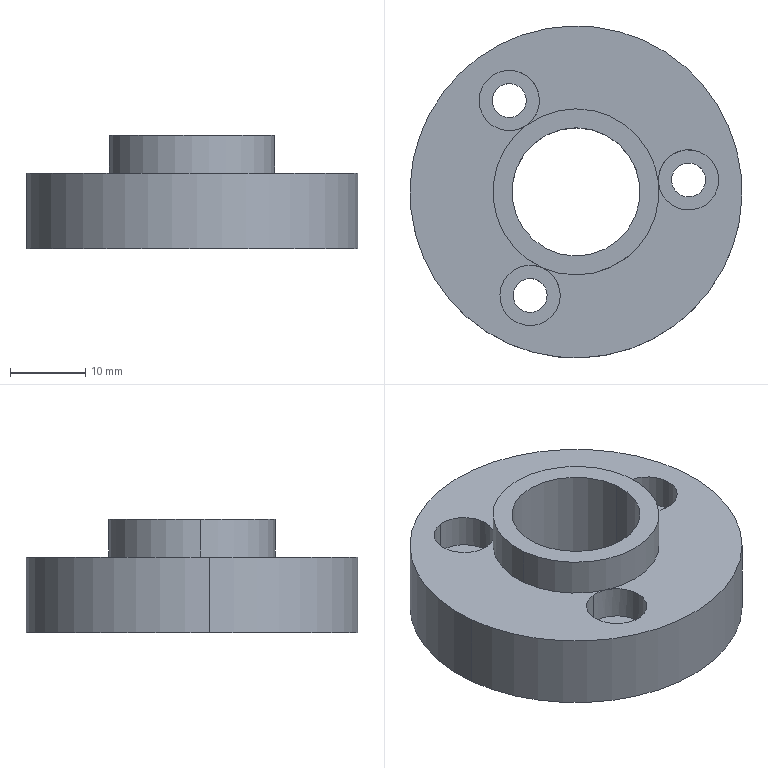Component | SolidWorks | XT-1-15-2-2 | 1 solid | 24 faces | box 44 x 44 x 15 mm | volume 12771 mm3 | cylinder 18 | plane 6 | commonest cylinder face diameters 8 x6 4.5 x6 17 x2 22 x2 44 x2
STEP:
#1=COLOUR_RGB('',0.7922,0.8196,0.9333);
#2=FILL_AREA_STYLE_COLOUR('',#1);
#3=FILL_AREA_STYLE('',(#2));
#4=SURFACE_STYLE_FILL_AREA(#3);
#5=SURFACE_SIDE_STYLE('',(#4));
#6=SURFACE_STYLE_USAGE(.BOTH.,#5);
#7=PRESENTATION_STYLE_ASSIGNMENT((#6));
#8=CARTESIAN_POINT('',(19.42,-9.62,-0.05512));
#9=VERTEX_POINT('',#8);
#10=CARTESIAN_POINT('',(19.454,-9.933,-0.05512));
#11=VERTEX_POINT('',#10);
#12=CARTESIAN_POINT('',(19.437,-9.777,-0.05512));
#13=DIRECTION('',(-0.,-0.,1.));
#14=DIRECTION('',(0.1062,-0.9943,-0.));
#15=AXIS2_PLACEMENT_3D('',#12,#13,#14);
#16=CIRCLE('',#15,0.1575);
#17=EDGE_CURVE('',#9,#11,#16,.T.);
#18=ORIENTED_EDGE('',*,*,#17,.F.);
#19=CARTESIAN_POINT('',(19.42,-9.62,0.1181));
#20=VERTEX_POINT('',#19);
#21=CARTESIAN_POINT('',(19.42,-9.62,0.1181));
#22=DIRECTION('',(-0.,-0.,1.));
#23=VECTOR('',#22,39.37);
#24=LINE('',#21,#23);
#25=EDGE_CURVE('',#9,#20,#24,.T.);
#26=ORIENTED_EDGE('',*,*,#25,.T.);
#27=CARTESIAN_POINT('',(19.454,-9.933,0.1181));
#28=VERTEX_POINT('',#27);
#29=CARTESIAN_POINT('',(19.437,-9.777,0.1181));
#30=DIRECTION('',(-0.,-0.,1.));
#31=DIRECTION('',(0.1062,-0.9943,-0.));
#32=AXIS2_PLACEMENT_3D('',#29,#30,#31);
#33=CIRCLE('',#32,0.1575);
#34=EDGE_CURVE('',#20,#28,#33,.T.);
#35=ORIENTED_EDGE('',*,*,#34,.T.);
#36=CARTESIAN_POINT('',(19.454,-9.933,0.1181));
#37=DIRECTION('',(-0.,-0.,1.));
#38=VECTOR('',#37,39.37);
#39=LINE('',#36,#38);
#40=EDGE_CURVE('',#11,#28,#39,.T.);
#41=ORIENTED_EDGE('',*,*,#40,.F.);
#42=EDGE_LOOP('',(#18,#26,#35,#41));
#43=FACE_OUTER_BOUND('',#42,.T.);
#44=CARTESIAN_POINT('',(19.437,-9.777,0.1181));
#45=DIRECTION('',(-0.,-0.,1.));
#46=DIRECTION('',(0.1062,-0.9943,-0.));
#47=AXIS2_PLACEMENT_3D('',#44,#45,#46);
#48=CYLINDRICAL_SURFACE('',#47,0.1575);
#49=ADVANCED_FACE('',(#43),#48,.F.);
#50=CARTESIAN_POINT('',(19.428,-9.689,-0.2756));
#51=VERTEX_POINT('',#50);
#52=CARTESIAN_POINT('',(19.447,-9.865,-0.2756));
#53=VERTEX_POINT('',#52);
#54=CARTESIAN_POINT('',(19.437,-9.777,-0.2756));
#55=DIRECTION('',(-0.,-0.,1.));
#56=DIRECTION('',(0.1062,-0.9943,0.));
#57=AXIS2_PLACEMENT_3D('',#54,#55,#56);
#58=CIRCLE('',#57,0.08858);
#59=EDGE_CURVE('',#51,#53,#58,.T.);
#60=ORIENTED_EDGE('',*,*,#59,.F.);
#61=CARTESIAN_POINT('',(19.428,-9.689,-0.05512));
#62=VERTEX_POINT('',#61);
#63=CARTESIAN_POINT('',(19.428,-9.689,0.1181));
#64=DIRECTION('',(-0.,-0.,1.));
#65=VECTOR('',#64,39.37);
#66=LINE('',#63,#65);
#67=EDGE_CURVE('',#51,#62,#66,.T.);
#68=ORIENTED_EDGE('',*,*,#67,.T.);
#69=CARTESIAN_POINT('',(19.447,-9.865,-0.05512));
#70=VERTEX_POINT('',#69);
#71=CARTESIAN_POINT('',(19.437,-9.777,-0.05512));
#72=DIRECTION('',(-0.,-0.,1.));
#73=DIRECTION('',(0.1062,-0.9943,-0.));
#74=AXIS2_PLACEMENT_3D('',#71,#72,#73);
#75=CIRCLE('',#74,0.08858);
#76=EDGE_CURVE('',#62,#70,#75,.T.);
#77=ORIENTED_EDGE('',*,*,#76,.T.);
#78=CARTESIAN_POINT('',(19.447,-9.865,0.1181));
#79=DIRECTION('',(-0.,-0.,1.));
#80=VECTOR('',#79,39.37);
#81=LINE('',#78,#80);
#82=EDGE_CURVE('',#53,#70,#81,.T.);
#83=ORIENTED_EDGE('',*,*,#82,.F.);
#84=EDGE_LOOP('',(#60,#68,#77,#83));
#85=FACE_OUTER_BOUND('',#84,.T.);
#86=CARTESIAN_POINT('',(19.437,-9.777,0.1181));
#87=DIRECTION('',(-0.,-0.,1.));
#88=DIRECTION('',(0.1062,-0.9943,0.));
#89=AXIS2_PLACEMENT_3D('',#86,#87,#88);
#90=CYLINDRICAL_SURFACE('',#89,0.08858);
#91=ADVANCED_FACE('',(#85),#90,.F.);
#92=CARTESIAN_POINT('',(19.312,-8.603,-0.05512));
#93=VERTEX_POINT('',#92);
#94=CARTESIAN_POINT('',(19.345,-8.916,-0.05512));
#95=VERTEX_POINT('',#94);
#96=CARTESIAN_POINT('',(19.329,-8.76,-0.05512));
#97=DIRECTION('',(-0.,-0.,1.));
#98=DIRECTION('',(0.1062,-0.9943,-0.));
#99=AXIS2_PLACEMENT_3D('',#96,#97,#98);
#100=CIRCLE('',#99,0.1575);
#101=EDGE_CURVE('',#93,#95,#100,.T.);
#102=ORIENTED_EDGE('',*,*,#101,.F.);
#103=CARTESIAN_POINT('',(19.312,-8.603,0.1181));
#104=VERTEX_POINT('',#103);
#105=CARTESIAN_POINT('',(19.312,-8.603,0.1181));
#106=DIRECTION('',(-0.,-0.,1.));
#107=VECTOR('',#106,39.37);
#108=LINE('',#105,#107);
#109=EDGE_CURVE('',#93,#104,#108,.T.);
#110=ORIENTED_EDGE('',*,*,#109,.T.);
#111=CARTESIAN_POINT('',(19.345,-8.916,0.1181));
#112=VERTEX_POINT('',#111);
#113=CARTESIAN_POINT('',(19.329,-8.76,0.1181));
#114=DIRECTION('',(-0.,-0.,1.));
#115=DIRECTION('',(0.1062,-0.9943,-0.));
#116=AXIS2_PLACEMENT_3D('',#113,#114,#115);
#117=CIRCLE('',#116,0.1575);
#118=EDGE_CURVE('',#104,#112,#117,.T.);
#119=ORIENTED_EDGE('',*,*,#118,.T.);
#120=CARTESIAN_POINT('',(19.345,-8.916,0.1181));
#121=DIRECTION('',(-0.,-0.,1.));
#122=VECTOR('',#121,39.37);
#123=LINE('',#120,#122);
#124=EDGE_CURVE('',#95,#112,#123,.T.);
#125=ORIENTED_EDGE('',*,*,#124,.F.);
#126=EDGE_LOOP('',(#102,#110,#119,#125));
#127=FACE_OUTER_BOUND('',#126,.T.);
#128=CARTESIAN_POINT('',(19.329,-8.76,0.1181));
#129=DIRECTION('',(-0.,-0.,1.));
#130=DIRECTION('',(0.1062,-0.9943,-0.));
#131=AXIS2_PLACEMENT_3D('',#128,#129,#130);
#132=CYLINDRICAL_SURFACE('',#131,0.1575);
#133=ADVANCED_FACE('',(#127),#132,.F.);
#134=CARTESIAN_POINT('',(19.319,-8.672,-0.2756));
#135=VERTEX_POINT('',#134);
#136=CARTESIAN_POINT('',(19.338,-8.848,-0.2756));
#137=VERTEX_POINT('',#136);
#138=CARTESIAN_POINT('',(19.329,-8.76,-0.2756));
#139=DIRECTION('',(-0.,-0.,1.));
#140=DIRECTION('',(0.1062,-0.9943,0.));
#141=AXIS2_PLACEMENT_3D('',#138,#139,#140);
#142=CIRCLE('',#141,0.08858);
#143=EDGE_CURVE('',#135,#137,#142,.T.);
#144=ORIENTED_EDGE('',*,*,#143,.F.);
#145=CARTESIAN_POINT('',(19.319,-8.672,-0.05512));
#146=VERTEX_POINT('',#145);
#147=CARTESIAN_POINT('',(19.319,-8.672,0.1181));
#148=DIRECTION('',(-0.,-0.,1.));
#149=VECTOR('',#148,39.37);
#150=LINE('',#147,#149);
#151=EDGE_CURVE('',#135,#146,#150,.T.);
#152=ORIENTED_EDGE('',*,*,#151,.T.);
#153=CARTESIAN_POINT('',(19.338,-8.848,-0.05512));
#154=VERTEX_POINT('',#153);
#155=CARTESIAN_POINT('',(19.329,-8.76,-0.05512));
#156=DIRECTION('',(-0.,-0.,1.));
#157=DIRECTION('',(0.1062,-0.9943,-0.));
#158=AXIS2_PLACEMENT_3D('',#155,#156,#157);
#159=CIRCLE('',#158,0.08858);
#160=EDGE_CURVE('',#146,#154,#159,.T.);
#161=ORIENTED_EDGE('',*,*,#160,.T.);
#162=CARTESIAN_POINT('',(19.338,-8.848,0.1181));
#163=DIRECTION('',(-0.,-0.,1.));
#164=VECTOR('',#163,39.37);
#165=LINE('',#162,#164);
#166=EDGE_CURVE('',#137,#154,#165,.T.);
#167=ORIENTED_EDGE('',*,*,#166,.F.);
#168=EDGE_LOOP('',(#144,#152,#161,#167));
#169=FACE_OUTER_BOUND('',#168,.T.);
#170=CARTESIAN_POINT('',(19.329,-8.76,0.1181));
#171=DIRECTION('',(-0.,-0.,1.));
#172=DIRECTION('',(0.1062,-0.9943,-0.));
#173=AXIS2_PLACEMENT_3D('',#170,#171,#172);
#174=CYLINDRICAL_SURFACE('',#173,0.08858);
#175=ADVANCED_FACE('',(#169),#174,.F.);
#176=CARTESIAN_POINT('',(20.247,-9.018,-0.05512));
#177=VERTEX_POINT('',#176);
#178=CARTESIAN_POINT('',(20.28,-9.331,-0.05512));
#179=VERTEX_POINT('',#178);
#180=CARTESIAN_POINT('',(20.264,-9.174,-0.05512));
#181=DIRECTION('',(-0.,-0.,1.));
#182=DIRECTION('',(0.1062,-0.9943,-0.));
#183=AXIS2_PLACEMENT_3D('',#180,#181,#182);
#184=CIRCLE('',#183,0.1575);
#185=EDGE_CURVE('',#177,#179,#184,.T.);
#186=ORIENTED_EDGE('',*,*,#185,.F.);
#187=CARTESIAN_POINT('',(20.247,-9.018,0.1181));
#188=VERTEX_POINT('',#187);
#189=CARTESIAN_POINT('',(20.247,-9.018,0.1181));
#190=DIRECTION('',(-0.,-0.,1.));
#191=VECTOR('',#190,39.37);
#192=LINE('',#189,#191);
#193=EDGE_CURVE('',#177,#188,#192,.T.);
#194=ORIENTED_EDGE('',*,*,#193,.T.);
#195=CARTESIAN_POINT('',(20.107,-9.191,0.1181));
#196=VERTEX_POINT('',#195);
#197=CARTESIAN_POINT('',(20.264,-9.174,0.1181));
#198=DIRECTION('',(-0.,-0.,1.));
#199=DIRECTION('',(0.1062,-0.9943,-0.));
#200=AXIS2_PLACEMENT_3D('',#197,#198,#199);
#201=CIRCLE('',#200,0.1575);
#202=EDGE_CURVE('',#188,#196,#201,.T.);
#203=ORIENTED_EDGE('',*,*,#202,.T.);
#204=CARTESIAN_POINT('',(20.28,-9.331,0.1181));
#205=VERTEX_POINT('',#204);
#206=CARTESIAN_POINT('',(20.264,-9.174,0.1181));
#207=DIRECTION('',(-0.,-0.,1.));
#208=DIRECTION('',(0.1062,-0.9943,-0.));
#209=AXIS2_PLACEMENT_3D('',#206,#207,#208);
#210=CIRCLE('',#209,0.1575);
#211=EDGE_CURVE('',#196,#205,#210,.T.);
#212=ORIENTED_EDGE('',*,*,#211,.T.);
#213=CARTESIAN_POINT('',(20.28,-9.331,0.1181));
#214=DIRECTION('',(-0.,-0.,1.));
#215=VECTOR('',#214,39.37);
#216=LINE('',#213,#215);
#217=EDGE_CURVE('',#179,#205,#216,.T.);
#218=ORIENTED_EDGE('',*,*,#217,.F.);
#219=EDGE_LOOP('',(#186,#194,#203,#212,#218));
#220=FACE_OUTER_BOUND('',#219,.T.);
#221=CARTESIAN_POINT('',(20.264,-9.174,0.1181));
#222=DIRECTION('',(-0.,-0.,1.));
#223=DIRECTION('',(0.1062,-0.9943,-0.));
#224=AXIS2_PLACEMENT_3D('',#221,#222,#223);
#225=CYLINDRICAL_SURFACE('',#224,0.1575);
#226=ADVANCED_FACE('',(#220),#225,.F.);
#227=CARTESIAN_POINT('',(20.254,-9.086,-0.2756));
#228=VERTEX_POINT('',#227);
#229=CARTESIAN_POINT('',(20.273,-9.262,-0.2756));
#230=VERTEX_POINT('',#229);
#231=CARTESIAN_POINT('',(20.264,-9.174,-0.2756));
#232=DIRECTION('',(-0.,-0.,1.));
#233=DIRECTION('',(0.1062,-0.9943,0.));
#234=AXIS2_PLACEMENT_3D('',#231,#232,#233);
#235=CIRCLE('',#234,0.08858);
#236=EDGE_CURVE('',#228,#230,#235,.T.);
#237=ORIENTED_EDGE('',*,*,#236,.F.);
#238=CARTESIAN_POINT('',(20.254,-9.086,-0.05512));
#239=VERTEX_POINT('',#238);
#240=CARTESIAN_POINT('',(20.254,-9.086,0.1181));
#241=DIRECTION('',(-0.,-0.,1.));
#242=VECTOR('',#241,39.37);
#243=LINE('',#240,#242);
#244=EDGE_CURVE('',#228,#239,#243,.T.);
#245=ORIENTED_EDGE('',*,*,#244,.T.);
#246=CARTESIAN_POINT('',(20.273,-9.262,-0.05512));
#247=VERTEX_POINT('',#246);
#248=CARTESIAN_POINT('',(20.264,-9.174,-0.05512));
#249=DIRECTION('',(-0.,-0.,1.));
#250=DIRECTION('',(0.1062,-0.9943,-0.));
#251=AXIS2_PLACEMENT_3D('',#248,#249,#250);
#252=CIRCLE('',#251,0.08858);
#253=EDGE_CURVE('',#239,#247,#252,.T.);
#254=ORIENTED_EDGE('',*,*,#253,.T.);
#255=CARTESIAN_POINT('',(20.273,-9.262,0.1181));
#256=DIRECTION('',(-0.,-0.,1.));
#257=VECTOR('',#256,39.37);
#258=LINE('',#255,#257);
#259=EDGE_CURVE('',#230,#247,#258,.T.);
#260=ORIENTED_EDGE('',*,*,#259,.F.);
#261=EDGE_LOOP('',(#237,#245,#254,#260));
#262=FACE_OUTER_BOUND('',#261,.T.);
#263=CARTESIAN_POINT('',(20.264,-9.174,0.1181));
#264=DIRECTION('',(-0.,-0.,1.));
#265=DIRECTION('',(0.1062,-0.9943,0.));
#266=AXIS2_PLACEMENT_3D('',#263,#264,#265);
#267=CYLINDRICAL_SURFACE('',#266,0.08858);
#268=ADVANCED_FACE('',(#262),#267,.F.);
#269=CARTESIAN_POINT('',(20.009,-9.201,-0.2756));
#270=VERTEX_POINT('',#269);
#271=CARTESIAN_POINT('',(19.344,-9.272,-0.2756));
#272=VERTEX_POINT('',#271);
#273=CARTESIAN_POINT('',(19.677,-9.237,-0.2756));
#274=DIRECTION('',(-0.,-0.,1.));
#275=DIRECTION('',(-0.9943,-0.1062,-0.));
#276=AXIS2_PLACEMENT_3D('',#273,#274,#275);
#277=CIRCLE('',#276,0.3346);
#278=EDGE_CURVE('',#270,#272,#277,.T.);
#279=ORIENTED_EDGE('',*,*,#278,.F.);
#280=CARTESIAN_POINT('',(20.009,-9.201,0.315));
#281=VERTEX_POINT('',#280);
#282=CARTESIAN_POINT('',(20.009,-9.201,-0.2756));
#283=DIRECTION('',(-0.,-0.,1.));
#284=VECTOR('',#283,39.37);
#285=LINE('',#282,#284);
#286=EDGE_CURVE('',#270,#281,#285,.T.);
#287=ORIENTED_EDGE('',*,*,#286,.T.);
#288=CARTESIAN_POINT('',(19.344,-9.272,0.315));
#289=VERTEX_POINT('',#288);
#290=CARTESIAN_POINT('',(19.677,-9.237,0.315));
#291=DIRECTION('',(-0.,-0.,1.));
#292=DIRECTION('',(-0.9943,-0.1062,-0.));
#293=AXIS2_PLACEMENT_3D('',#290,#291,#292);
#294=CIRCLE('',#293,0.3346);
#295=EDGE_CURVE('',#281,#289,#294,.T.);
#296=ORIENTED_EDGE('',*,*,#295,.T.);
#297=CARTESIAN_POINT('',(19.344,-9.272,-0.2756));
#298=DIRECTION('',(-0.,-0.,1.));
#299=VECTOR('',#298,39.37);
#300=LINE('',#297,#299);
#301=EDGE_CURVE('',#272,#289,#300,.T.);
#302=ORIENTED_EDGE('',*,*,#301,.F.);
#303=EDGE_LOOP('',(#279,#287,#296,#302));
#304=FACE_OUTER_BOUND('',#303,.T.);
#305=CARTESIAN_POINT('',(19.677,-9.237,-0.2756));
#306=DIRECTION('',(-0.,-0.,1.));
#307=DIRECTION('',(-0.9943,-0.1062,-0.));
#308=AXIS2_PLACEMENT_3D('',#305,#306,#307);
#309=CYLINDRICAL_SURFACE('',#308,0.3346);
#310=ADVANCED_FACE('',(#304),#309,.F.);
#311=CARTESIAN_POINT('',(19.501,-9.633,0.1181));
#312=VERTEX_POINT('',#311);
#313=CARTESIAN_POINT('',(19.677,-9.237,0.1181));
#314=DIRECTION('',(-0.,-0.,1.));
#315=DIRECTION('',(-0.9943,-0.1062,-0.));
#316=AXIS2_PLACEMENT_3D('',#313,#314,#315);
#317=CIRCLE('',#316,0.4331);
#318=EDGE_CURVE('',#312,#196,#317,.T.);
#319=ORIENTED_EDGE('',*,*,#318,.T.);
#320=CARTESIAN_POINT('',(20.107,-9.191,0.315));
#321=VERTEX_POINT('',#320);
#322=CARTESIAN_POINT('',(20.107,-9.191,0.315));
#323=DIRECTION('',(-0.,-0.,1.));
#324=VECTOR('',#323,39.37);
#325=LINE('',#322,#324);
#326=EDGE_CURVE('',#196,#321,#325,.T.);
#327=ORIENTED_EDGE('',*,*,#326,.T.);
#328=CARTESIAN_POINT('',(19.246,-9.283,0.315));
#329=VERTEX_POINT('',#328);
#330=CARTESIAN_POINT('',(19.677,-9.237,0.315));
#331=DIRECTION('',(-0.,-0.,1.));
#332=DIRECTION('',(-0.9943,-0.1062,-0.));
#333=AXIS2_PLACEMENT_3D('',#330,#331,#332);
#334=CIRCLE('',#333,0.4331);
#335=EDGE_CURVE('',#329,#321,#334,.T.);
#336=ORIENTED_EDGE('',*,*,#335,.F.);
#337=CARTESIAN_POINT('',(19.246,-9.283,0.1181));
#338=VERTEX_POINT('',#337);
#339=CARTESIAN_POINT('',(19.246,-9.283,0.315));
#340=DIRECTION('',(-0.,-0.,1.));
#341=VECTOR('',#340,39.37);
#342=LINE('',#339,#341);
#343=EDGE_CURVE('',#338,#329,#342,.T.);
#344=ORIENTED_EDGE('',*,*,#343,.F.);
#345=CARTESIAN_POINT('',(19.677,-9.237,0.1181));
#346=DIRECTION('',(-0.,-0.,1.));
#347=DIRECTION('',(-0.9943,-0.1062,-0.));
#348=AXIS2_PLACEMENT_3D('',#345,#346,#347);
#349=CIRCLE('',#348,0.4331);
#350=EDGE_CURVE('',#338,#312,#349,.T.);
#351=ORIENTED_EDGE('',*,*,#350,.T.);
#352=EDGE_LOOP('',(#319,#327,#336,#344,#351));
#353=FACE_OUTER_BOUND('',#352,.T.);
#354=CARTESIAN_POINT('',(19.677,-9.237,0.315));
#355=DIRECTION('',(-0.,-0.,1.));
#356=DIRECTION('',(-0.9943,-0.1062,-0.));
#357=AXIS2_PLACEMENT_3D('',#354,#355,#356);
#358=CYLINDRICAL_SURFACE('',#357,0.4331);
#359=ADVANCED_FACE('',(#353),#358,.T.);
#360=CARTESIAN_POINT('',(18.815,-9.329,-0.2756));
#361=VERTEX_POINT('',#360);
#362=CARTESIAN_POINT('',(20.538,-9.145,-0.2756));
#363=VERTEX_POINT('',#362);
#364=CARTESIAN_POINT('',(19.677,-9.237,-0.2756));
#365=DIRECTION('',(-0.,-0.,1.));
#366=DIRECTION('',(-0.9943,-0.1062,-0.));
#367=AXIS2_PLACEMENT_3D('',#364,#365,#366);
#368=CIRCLE('',#367,0.8661);
#369=EDGE_CURVE('',#361,#363,#368,.T.);
#370=ORIENTED_EDGE('',*,*,#369,.T.);
#371=CARTESIAN_POINT('',(20.538,-9.145,0.1181));
#372=VERTEX_POINT('',#371);
#373=CARTESIAN_POINT('',(20.538,-9.145,0.315));
#374=DIRECTION('',(-0.,-0.,1.));
#375=VECTOR('',#374,39.37);
#376=LINE('',#373,#375);
#377=EDGE_CURVE('',#363,#372,#376,.T.);
#378=ORIENTED_EDGE('',*,*,#377,.T.);
#379=CARTESIAN_POINT('',(18.815,-9.329,0.1181));
#380=VERTEX_POINT('',#379);
#381=CARTESIAN_POINT('',(19.677,-9.237,0.1181));
#382=DIRECTION('',(-0.,-0.,1.));
#383=DIRECTION('',(-0.9943,-0.1062,-0.));
#384=AXIS2_PLACEMENT_3D('',#381,#382,#383);
#385=CIRCLE('',#384,0.8661);
#386=EDGE_CURVE('',#380,#372,#385,.T.);
#387=ORIENTED_EDGE('',*,*,#386,.F.);
#388=CARTESIAN_POINT('',(18.815,-9.329,0.315));
#389=DIRECTION('',(-0.,-0.,1.));
#390=VECTOR('',#389,39.37);
#391=LINE('',#388,#390);
#392=EDGE_CURVE('',#361,#380,#391,.T.);
#393=ORIENTED_EDGE('',*,*,#392,.F.);
#394=EDGE_LOOP('',(#370,#378,#387,#393));
#395=FACE_OUTER_BOUND('',#394,.T.);
#396=CARTESIAN_POINT('',(19.677,-9.237,0.315));
#397=DIRECTION('',(-0.,-0.,1.));
#398=DIRECTION('',(-0.9943,-0.1062,-0.));
#399=AXIS2_PLACEMENT_3D('',#396,#397,#398);
#400=CYLINDRICAL_SURFACE('',#399,0.8661);
#401=ADVANCED_FACE('',(#395),#400,.T.);
#402=ORIENTED_EDGE('',*,*,#386,.T.);
#403=CARTESIAN_POINT('',(19.677,-9.237,0.1181));
#404=DIRECTION('',(-0.,-0.,1.));
#405=DIRECTION('',(-0.9943,-0.1062,-0.));
#406=AXIS2_PLACEMENT_3D('',#403,#404,#405);
#407=CIRCLE('',#406,0.8661);
#408=EDGE_CURVE('',#372,#380,#407,.T.);
#409=ORIENTED_EDGE('',*,*,#408,.T.);
#410=EDGE_LOOP('',(#402,#409));
#411=FACE_OUTER_BOUND('',#410,.T.);
#412=ORIENTED_EDGE('',*,*,#318,.F.);
#413=CARTESIAN_POINT('',(19.437,-9.777,0.1181));
#414=DIRECTION('',(-0.,-0.,1.));
#415=DIRECTION('',(0.1062,-0.9943,-0.));
#416=AXIS2_PLACEMENT_3D('',#413,#414,#415);
#417=CIRCLE('',#416,0.1575);
#418=EDGE_CURVE('',#28,#312,#417,.T.);
#419=ORIENTED_EDGE('',*,*,#418,.F.);
#420=ORIENTED_EDGE('',*,*,#34,.F.);
#421=CARTESIAN_POINT('',(19.437,-9.777,0.1181));
#422=DIRECTION('',(-0.,-0.,1.));
#423=DIRECTION('',(0.1062,-0.9943,-0.));
#424=AXIS2_PLACEMENT_3D('',#421,#422,#423);
#425=CIRCLE('',#424,0.1575);
#426=EDGE_CURVE('',#312,#20,#425,.T.);
#427=ORIENTED_EDGE('',*,*,#426,.F.);
#428=ORIENTED_EDGE('',*,*,#350,.F.);
#429=CARTESIAN_POINT('',(19.421,-8.887,0.1181));
#430=VERTEX_POINT('',#429);
#431=CARTESIAN_POINT('',(19.677,-9.237,0.1181));
#432=DIRECTION('',(-0.,-0.,1.));
#433=DIRECTION('',(-0.9943,-0.1062,-0.));
#434=AXIS2_PLACEMENT_3D('',#431,#432,#433);
#435=CIRCLE('',#434,0.4331);
#436=EDGE_CURVE('',#430,#338,#435,.T.);
#437=ORIENTED_EDGE('',*,*,#436,.F.);
#438=CARTESIAN_POINT('',(19.329,-8.76,0.1181));
#439=DIRECTION('',(-0.,-0.,1.));
#440=DIRECTION('',(0.1062,-0.9943,-0.));
#441=AXIS2_PLACEMENT_3D('',#438,#439,#440);
#442=CIRCLE('',#441,0.1575);
#443=EDGE_CURVE('',#112,#430,#442,.T.);
#444=ORIENTED_EDGE('',*,*,#443,.F.);
#445=ORIENTED_EDGE('',*,*,#118,.F.);
#446=CARTESIAN_POINT('',(19.329,-8.76,0.1181));
#447=DIRECTION('',(-0.,-0.,1.));
#448=DIRECTION('',(0.1062,-0.9943,-0.));
#449=AXIS2_PLACEMENT_3D('',#446,#447,#448);
#450=CIRCLE('',#449,0.1575);
#451=EDGE_CURVE('',#430,#104,#450,.T.);
#452=ORIENTED_EDGE('',*,*,#451,.F.);
#453=CARTESIAN_POINT('',(19.677,-9.237,0.1181));
#454=DIRECTION('',(-0.,-0.,1.));
#455=DIRECTION('',(-0.9943,-0.1062,-0.));
#456=AXIS2_PLACEMENT_3D('',#453,#454,#455);
#457=CIRCLE('',#456,0.4331);
#458=EDGE_CURVE('',#196,#430,#457,.T.);
#459=ORIENTED_EDGE('',*,*,#458,.F.);
#460=ORIENTED_EDGE('',*,*,#202,.F.);
#461=CARTESIAN_POINT('',(20.264,-9.174,0.1181));
#462=DIRECTION('',(-0.,-0.,1.));
#463=DIRECTION('',(0.1062,-0.9943,-0.));
#464=AXIS2_PLACEMENT_3D('',#461,#462,#463);
#465=CIRCLE('',#464,0.1575);
#466=EDGE_CURVE('',#205,#188,#465,.T.);
#467=ORIENTED_EDGE('',*,*,#466,.F.);
#468=ORIENTED_EDGE('',*,*,#211,.F.);
#469=EDGE_LOOP('',(#412,#419,#420,#427,#428,#437,#444,#445,#452,#459,#460,#467,#468));
#470=FACE_BOUND('',#469,.T.);
#471=CARTESIAN_POINT('',(20.538,-9.145,0.1181));
#472=DIRECTION('',(0.,0.,-1.));
#473=DIRECTION('',(0.9943,0.1062,0.));
#474=AXIS2_PLACEMENT_3D('',#471,#472,#473);
#475=PLANE('',#474);
#476=ADVANCED_FACE('',(#411,#470),#475,.F.);
#477=CARTESIAN_POINT('',(19.677,-9.237,0.315));
#478=DIRECTION('',(-0.,-0.,1.));
#479=DIRECTION('',(-0.9943,-0.1062,-0.));
#480=AXIS2_PLACEMENT_3D('',#477,#478,#479);
#481=CIRCLE('',#480,0.3346);
#482=EDGE_CURVE('',#289,#281,#481,.T.);
#483=ORIENTED_EDGE('',*,*,#482,.F.);
#484=ORIENTED_EDGE('',*,*,#295,.F.);
#485=EDGE_LOOP('',(#483,#484));
#486=FACE_BOUND('',#485,.T.);
#487=ORIENTED_EDGE('',*,*,#335,.T.);
#488=CARTESIAN_POINT('',(19.677,-9.237,0.315));
#489=DIRECTION('',(-0.,-0.,1.));
#490=DIRECTION('',(-0.9943,-0.1062,-0.));
#491=AXIS2_PLACEMENT_3D('',#488,#489,#490);
#492=CIRCLE('',#491,0.4331);
#493=EDGE_CURVE('',#321,#329,#492,.T.);
#494=ORIENTED_EDGE('',*,*,#493,.T.);
#495=EDGE_LOOP('',(#487,#494));
#496=FACE_OUTER_BOUND('',#495,.T.);
#497=CARTESIAN_POINT('',(20.107,-9.191,0.315));
#498=DIRECTION('',(0.,0.,-1.));
#499=DIRECTION('',(0.9943,0.1062,0.));
#500=AXIS2_PLACEMENT_3D('',#497,#498,#499);
#501=PLANE('',#500);
#502=ADVANCED_FACE('',(#486,#496),#501,.F.);
#503=CARTESIAN_POINT('',(19.437,-9.777,-0.2756));
#504=DIRECTION('',(-0.,-0.,1.));
#505=DIRECTION('',(0.1062,-0.9943,0.));
#506=AXIS2_PLACEMENT_3D('',#503,#504,#505);
#507=CIRCLE('',#506,0.08858);
#508=EDGE_CURVE('',#53,#51,#507,.T.);
#509=ORIENTED_EDGE('',*,*,#508,.T.);
#510=ORIENTED_EDGE('',*,*,#59,.T.);
#511=EDGE_LOOP('',(#509,#510));
#512=FACE_BOUND('',#511,.T.);
#513=CARTESIAN_POINT('',(19.329,-8.76,-0.2756));
#514=DIRECTION('',(-0.,-0.,1.));
#515=DIRECTION('',(0.1062,-0.9943,0.));
#516=AXIS2_PLACEMENT_3D('',#513,#514,#515);
#517=CIRCLE('',#516,0.08858);
#518=EDGE_CURVE('',#137,#135,#517,.T.);
#519=ORIENTED_EDGE('',*,*,#518,.T.);
#520=ORIENTED_EDGE('',*,*,#143,.T.);
#521=EDGE_LOOP('',(#519,#520));
#522=FACE_BOUND('',#521,.T.);
#523=CARTESIAN_POINT('',(20.264,-9.174,-0.2756));
#524=DIRECTION('',(-0.,-0.,1.));
#525=DIRECTION('',(0.1062,-0.9943,0.));
#526=AXIS2_PLACEMENT_3D('',#523,#524,#525);
#527=CIRCLE('',#526,0.08858);
#528=EDGE_CURVE('',#230,#228,#527,.T.);
#529=ORIENTED_EDGE('',*,*,#528,.T.);
#530=ORIENTED_EDGE('',*,*,#236,.T.);
#531=EDGE_LOOP('',(#529,#530));
#532=FACE_BOUND('',#531,.T.);
#533=CARTESIAN_POINT('',(19.677,-9.237,-0.2756));
#534=DIRECTION('',(-0.,-0.,1.));
#535=DIRECTION('',(-0.9943,-0.1062,-0.));
#536=AXIS2_PLACEMENT_3D('',#533,#534,#535);
#537=CIRCLE('',#536,0.3346);
#538=EDGE_CURVE('',#272,#270,#537,.T.);
#539=ORIENTED_EDGE('',*,*,#538,.T.);
#540=ORIENTED_EDGE('',*,*,#278,.T.);
#541=EDGE_LOOP('',(#539,#540));
#542=FACE_BOUND('',#541,.T.);
#543=ORIENTED_EDGE('',*,*,#369,.F.);
#544=CARTESIAN_POINT('',(19.677,-9.237,-0.2756));
#545=DIRECTION('',(-0.,-0.,1.));
#546=DIRECTION('',(-0.9943,-0.1062,-0.));
#547=AXIS2_PLACEMENT_3D('',#544,#545,#546);
#548=CIRCLE('',#547,0.8661);
#549=EDGE_CURVE('',#363,#361,#548,.T.);
#550=ORIENTED_EDGE('',*,*,#549,.F.);
#551=EDGE_LOOP('',(#543,#550));
#552=FACE_OUTER_BOUND('',#551,.T.);
#553=CARTESIAN_POINT('',(19.677,-9.237,-0.2756));
#554=DIRECTION('',(-0.,-0.,1.));
#555=DIRECTION('',(-0.9943,-0.1062,-0.));
#556=AXIS2_PLACEMENT_3D('',#553,#554,#555);
#557=PLANE('',#556);
#558=ADVANCED_FACE('',(#512,#522,#532,#542,#552),#557,.F.);
#559=ORIENTED_EDGE('',*,*,#377,.F.);
#560=ORIENTED_EDGE('',*,*,#549,.T.);
#561=ORIENTED_EDGE('',*,*,#392,.T.);
#562=ORIENTED_EDGE('',*,*,#408,.F.);
#563=EDGE_LOOP('',(#559,#560,#561,#562));
#564=FACE_OUTER_BOUND('',#563,.T.);
#565=CARTESIAN_POINT('',(19.677,-9.237,0.315));
#566=DIRECTION('',(-0.,-0.,1.));
#567=DIRECTION('',(-0.9943,-0.1062,-0.));
#568=AXIS2_PLACEMENT_3D('',#565,#566,#567);
#569=CYLINDRICAL_SURFACE('',#568,0.8661);
#570=ADVANCED_FACE('',(#564),#569,.T.);
#571=ORIENTED_EDGE('',*,*,#326,.F.);
#572=ORIENTED_EDGE('',*,*,#458,.T.);
#573=ORIENTED_EDGE('',*,*,#436,.T.);
#574=ORIENTED_EDGE('',*,*,#343,.T.);
#575=ORIENTED_EDGE('',*,*,#493,.F.);
#576=EDGE_LOOP('',(#571,#572,#573,#574,#575));
#577=FACE_OUTER_BOUND('',#576,.T.);
#578=CARTESIAN_POINT('',(19.677,-9.237,0.315));
#579=DIRECTION('',(-0.,-0.,1.));
#580=DIRECTION('',(-0.9943,-0.1062,-0.));
#581=AXIS2_PLACEMENT_3D('',#578,#579,#580);
#582=CYLINDRICAL_SURFACE('',#581,0.4331);
#583=ADVANCED_FACE('',(#577),#582,.T.);
#584=ORIENTED_EDGE('',*,*,#286,.F.);
#585=ORIENTED_EDGE('',*,*,#538,.F.);
#586=ORIENTED_EDGE('',*,*,#301,.T.);
#587=ORIENTED_EDGE('',*,*,#482,.T.);
#588=EDGE_LOOP('',(#584,#585,#586,#587));
#589=FACE_OUTER_BOUND('',#588,.T.);
#590=CARTESIAN_POINT('',(19.677,-9.237,-0.2756));
#591=DIRECTION('',(-0.,-0.,1.));
#592=DIRECTION('',(-0.9943,-0.1062,-0.));
#593=AXIS2_PLACEMENT_3D('',#590,#591,#592);
#594=CYLINDRICAL_SURFACE('',#593,0.3346);
#595=ADVANCED_FACE('',(#589),#594,.F.);
#596=ORIENTED_EDGE('',*,*,#244,.F.);
#597=ORIENTED_EDGE('',*,*,#528,.F.);
#598=ORIENTED_EDGE('',*,*,#259,.T.);
#599=CARTESIAN_POINT('',(20.264,-9.174,-0.05512));
#600=DIRECTION('',(-0.,-0.,1.));
#601=DIRECTION('',(0.1062,-0.9943,-0.));
#602=AXIS2_PLACEMENT_3D('',#599,#600,#601);
#603=CIRCLE('',#602,0.08858);
#604=EDGE_CURVE('',#247,#239,#603,.T.);
#605=ORIENTED_EDGE('',*,*,#604,.T.);
#606=EDGE_LOOP('',(#596,#597,#598,#605));
#607=FACE_OUTER_BOUND('',#606,.T.);
#608=CARTESIAN_POINT('',(20.264,-9.174,0.1181));
#609=DIRECTION('',(-0.,-0.,1.));
#610=DIRECTION('',(0.1062,-0.9943,0.));
#611=AXIS2_PLACEMENT_3D('',#608,#609,#610);
#612=CYLINDRICAL_SURFACE('',#611,0.08858);
#613=ADVANCED_FACE('',(#607),#612,.F.);
#614=ORIENTED_EDGE('',*,*,#604,.F.);
#615=ORIENTED_EDGE('',*,*,#253,.F.);
#616=EDGE_LOOP('',(#614,#615));
#617=FACE_BOUND('',#616,.T.);
#618=CARTESIAN_POINT('',(20.264,-9.174,-0.05512));
#619=DIRECTION('',(-0.,-0.,1.));
#620=DIRECTION('',(0.1062,-0.9943,-0.));
#621=AXIS2_PLACEMENT_3D('',#618,#619,#620);
#622=CIRCLE('',#621,0.1575);
#623=EDGE_CURVE('',#179,#177,#622,.T.);
#624=ORIENTED_EDGE('',*,*,#623,.T.);
#625=ORIENTED_EDGE('',*,*,#185,.T.);
#626=EDGE_LOOP('',(#624,#625));
#627=FACE_OUTER_BOUND('',#626,.T.);
#628=CARTESIAN_POINT('',(20.352,-9.165,-0.05512));
#629=DIRECTION('',(0.,0.,-1.));
#630=DIRECTION('',(-0.1062,0.9943,0.));
#631=AXIS2_PLACEMENT_3D('',#628,#629,#630);
#632=PLANE('',#631);
#633=ADVANCED_FACE('',(#617,#627),#632,.F.);
#634=ORIENTED_EDGE('',*,*,#193,.F.);
#635=ORIENTED_EDGE('',*,*,#623,.F.);
#636=ORIENTED_EDGE('',*,*,#217,.T.);
#637=ORIENTED_EDGE('',*,*,#466,.T.);
#638=EDGE_LOOP('',(#634,#635,#636,#637));
#639=FACE_OUTER_BOUND('',#638,.T.);
#640=CARTESIAN_POINT('',(20.264,-9.174,0.1181));
#641=DIRECTION('',(-0.,-0.,1.));
#642=DIRECTION('',(0.1062,-0.9943,-0.));
#643=AXIS2_PLACEMENT_3D('',#640,#641,#642);
#644=CYLINDRICAL_SURFACE('',#643,0.1575);
#645=ADVANCED_FACE('',(#639),#644,.F.);
#646=ORIENTED_EDGE('',*,*,#151,.F.);
#647=ORIENTED_EDGE('',*,*,#518,.F.);
#648=ORIENTED_EDGE('',*,*,#166,.T.);
#649=CARTESIAN_POINT('',(19.329,-8.76,-0.05512));
#650=DIRECTION('',(-0.,-0.,1.));
#651=DIRECTION('',(0.1062,-0.9943,-0.));
#652=AXIS2_PLACEMENT_3D('',#649,#650,#651);
#653=CIRCLE('',#652,0.08858);
#654=EDGE_CURVE('',#154,#146,#653,.T.);
#655=ORIENTED_EDGE('',*,*,#654,.T.);
#656=EDGE_LOOP('',(#646,#647,#648,#655));
#657=FACE_OUTER_BOUND('',#656,.T.);
#658=CARTESIAN_POINT('',(19.329,-8.76,0.1181));
#659=DIRECTION('',(-0.,-0.,1.));
#660=DIRECTION('',(0.1062,-0.9943,-0.));
#661=AXIS2_PLACEMENT_3D('',#658,#659,#660);
#662=CYLINDRICAL_SURFACE('',#661,0.08858);
#663=ADVANCED_FACE('',(#657),#662,.F.);
#664=ORIENTED_EDGE('',*,*,#654,.F.);
#665=ORIENTED_EDGE('',*,*,#160,.F.);
#666=EDGE_LOOP('',(#664,#665));
#667=FACE_BOUND('',#666,.T.);
#668=CARTESIAN_POINT('',(19.329,-8.76,-0.05512));
#669=DIRECTION('',(-0.,-0.,1.));
#670=DIRECTION('',(0.1062,-0.9943,-0.));
#671=AXIS2_PLACEMENT_3D('',#668,#669,#670);
#672=CIRCLE('',#671,0.1575);
#673=EDGE_CURVE('',#95,#93,#672,.T.);
#674=ORIENTED_EDGE('',*,*,#673,.T.);
#675=ORIENTED_EDGE('',*,*,#101,.T.);
#676=EDGE_LOOP('',(#674,#675));
#677=FACE_OUTER_BOUND('',#676,.T.);
#678=CARTESIAN_POINT('',(19.417,-8.75,-0.05512));
#679=DIRECTION('',(0.,0.,-1.));
#680=DIRECTION('',(-0.1062,0.9943,0.));
#681=AXIS2_PLACEMENT_3D('',#678,#679,#680);
#682=PLANE('',#681);
#683=ADVANCED_FACE('',(#667,#677),#682,.F.);
#684=ORIENTED_EDGE('',*,*,#109,.F.);
#685=ORIENTED_EDGE('',*,*,#673,.F.);
#686=ORIENTED_EDGE('',*,*,#124,.T.);
#687=ORIENTED_EDGE('',*,*,#443,.T.);
#688=ORIENTED_EDGE('',*,*,#451,.T.);
#689=EDGE_LOOP('',(#684,#685,#686,#687,#688));
#690=FACE_OUTER_BOUND('',#689,.T.);
#691=CARTESIAN_POINT('',(19.329,-8.76,0.1181));
#692=DIRECTION('',(-0.,-0.,1.));
#693=DIRECTION('',(0.1062,-0.9943,-0.));
#694=AXIS2_PLACEMENT_3D('',#691,#692,#693);
#695=CYLINDRICAL_SURFACE('',#694,0.1575);
#696=ADVANCED_FACE('',(#690),#695,.F.);
#697=ORIENTED_EDGE('',*,*,#67,.F.);
#698=ORIENTED_EDGE('',*,*,#508,.F.);
#699=ORIENTED_EDGE('',*,*,#82,.T.);
#700=CARTESIAN_POINT('',(19.437,-9.777,-0.05512));
#701=DIRECTION('',(-0.,-0.,1.));
#702=DIRECTION('',(0.1062,-0.9943,-0.));
#703=AXIS2_PLACEMENT_3D('',#700,#701,#702);
#704=CIRCLE('',#703,0.08858);
#705=EDGE_CURVE('',#70,#62,#704,.T.);
#706=ORIENTED_EDGE('',*,*,#705,.T.);
#707=EDGE_LOOP('',(#697,#698,#699,#706));
#708=FACE_OUTER_BOUND('',#707,.T.);
#709=CARTESIAN_POINT('',(19.437,-9.777,0.1181));
#710=DIRECTION('',(-0.,-0.,1.));
#711=DIRECTION('',(0.1062,-0.9943,0.));
#712=AXIS2_PLACEMENT_3D('',#709,#710,#711);
#713=CYLINDRICAL_SURFACE('',#712,0.08858);
#714=ADVANCED_FACE('',(#708),#713,.F.);
#715=ORIENTED_EDGE('',*,*,#705,.F.);
#716=ORIENTED_EDGE('',*,*,#76,.F.);
#717=EDGE_LOOP('',(#715,#716));
#718=FACE_BOUND('',#717,.T.);
#719=CARTESIAN_POINT('',(19.437,-9.777,-0.05512));
#720=DIRECTION('',(-0.,-0.,1.));
#721=DIRECTION('',(0.1062,-0.9943,-0.));
#722=AXIS2_PLACEMENT_3D('',#719,#720,#721);
#723=CIRCLE('',#722,0.1575);
#724=EDGE_CURVE('',#11,#9,#723,.T.);
#725=ORIENTED_EDGE('',*,*,#724,.T.);
#726=ORIENTED_EDGE('',*,*,#17,.T.);
#727=EDGE_LOOP('',(#725,#726));
#728=FACE_OUTER_BOUND('',#727,.T.);
#729=CARTESIAN_POINT('',(19.525,-9.767,-0.05512));
#730=DIRECTION('',(0.,0.,-1.));
#731=DIRECTION('',(-0.1062,0.9943,0.));
#732=AXIS2_PLACEMENT_3D('',#729,#730,#731);
#733=PLANE('',#732);
#734=ADVANCED_FACE('',(#718,#728),#733,.F.);
#735=ORIENTED_EDGE('',*,*,#25,.F.);
#736=ORIENTED_EDGE('',*,*,#724,.F.);
#737=ORIENTED_EDGE('',*,*,#40,.T.);
#738=ORIENTED_EDGE('',*,*,#418,.T.);
#739=ORIENTED_EDGE('',*,*,#426,.T.);
#740=EDGE_LOOP('',(#735,#736,#737,#738,#739));
#741=FACE_OUTER_BOUND('',#740,.T.);
#742=CARTESIAN_POINT('',(19.437,-9.777,0.1181));
#743=DIRECTION('',(-0.,-0.,1.));
#744=DIRECTION('',(0.1062,-0.9943,-0.));
#745=AXIS2_PLACEMENT_3D('',#742,#743,#744);
#746=CYLINDRICAL_SURFACE('',#745,0.1575);
#747=ADVANCED_FACE('',(#741),#746,.F.);
#748=CLOSED_SHELL('',(#49,#91,#133,#175,#226,#268,#310,#359,#401,#476,#502,#558,#570,#583,#595,#613,#633,#645,#663,#683,#696,#714,#734,#747));
#749=MANIFOLD_SOLID_BREP('',#748);
#750=STYLED_ITEM('',(#7),#749);
#751=PRESENTATION_LAYER_ASSIGNMENT('','',(#750));
#752=CARTESIAN_POINT('',(0.,0.,0.));
#753=DIRECTION('',(0.,0.,1.));
#754=DIRECTION('',(1.,0.,0.));
#755=AXIS2_PLACEMENT_3D('',#752,#753,#754);
#756=(LENGTH_UNIT()NAMED_UNIT(*)SI_UNIT($,.METRE.));
#757=LENGTH_MEASURE_WITH_UNIT(LENGTH_MEASURE(0.0254),#756);
#758=DIMENSIONAL_EXPONENTS(1.,0.,0.,0.,0.,0.,0.);
#759=(CONVERSION_BASED_UNIT('',#757)LENGTH_UNIT()NAMED_UNIT(#758));
#760=UNCERTAINTY_MEASURE_WITH_UNIT(LENGTH_MEASURE(0.00001),#759,'','');
#761=(NAMED_UNIT(*)PLANE_ANGLE_UNIT()SI_UNIT($,.RADIAN.));
#762=(NAMED_UNIT(*)SI_UNIT($,.STERADIAN.)SOLID_ANGLE_UNIT());
#763=(GEOMETRIC_REPRESENTATION_CONTEXT(3)GLOBAL_UNCERTAINTY_ASSIGNED_CONTEXT((#760))GLOBAL_UNIT_ASSIGNED_CONTEXT((#759,#761,#762))REPRESENTATION_CONTEXT('',''));
#764=ADVANCED_BREP_SHAPE_REPRESENTATION('',(#749,#755),#763);
#765=(LENGTH_UNIT()NAMED_UNIT(*)SI_UNIT($,.METRE.));
#766=LENGTH_MEASURE_WITH_UNIT(LENGTH_MEASURE(0.0254),#765);
#767=DIMENSIONAL_EXPONENTS(1.,0.,0.,0.,0.,0.,0.);
#768=(CONVERSION_BASED_UNIT('',#766)LENGTH_UNIT()NAMED_UNIT(#767));
#769=UNCERTAINTY_MEASURE_WITH_UNIT(LENGTH_MEASURE(0.00001),#768,'','');
#770=(NAMED_UNIT(*)PLANE_ANGLE_UNIT()SI_UNIT($,.RADIAN.));
#771=(NAMED_UNIT(*)SI_UNIT($,.STERADIAN.)SOLID_ANGLE_UNIT());
#772=(GEOMETRIC_REPRESENTATION_CONTEXT(3)GLOBAL_UNCERTAINTY_ASSIGNED_CONTEXT((#769))GLOBAL_UNIT_ASSIGNED_CONTEXT((#768,#770,#771))REPRESENTATION_CONTEXT('',''));
#773=MECHANICAL_DESIGN_GEOMETRIC_PRESENTATION_REPRESENTATION('',(#750),#772);